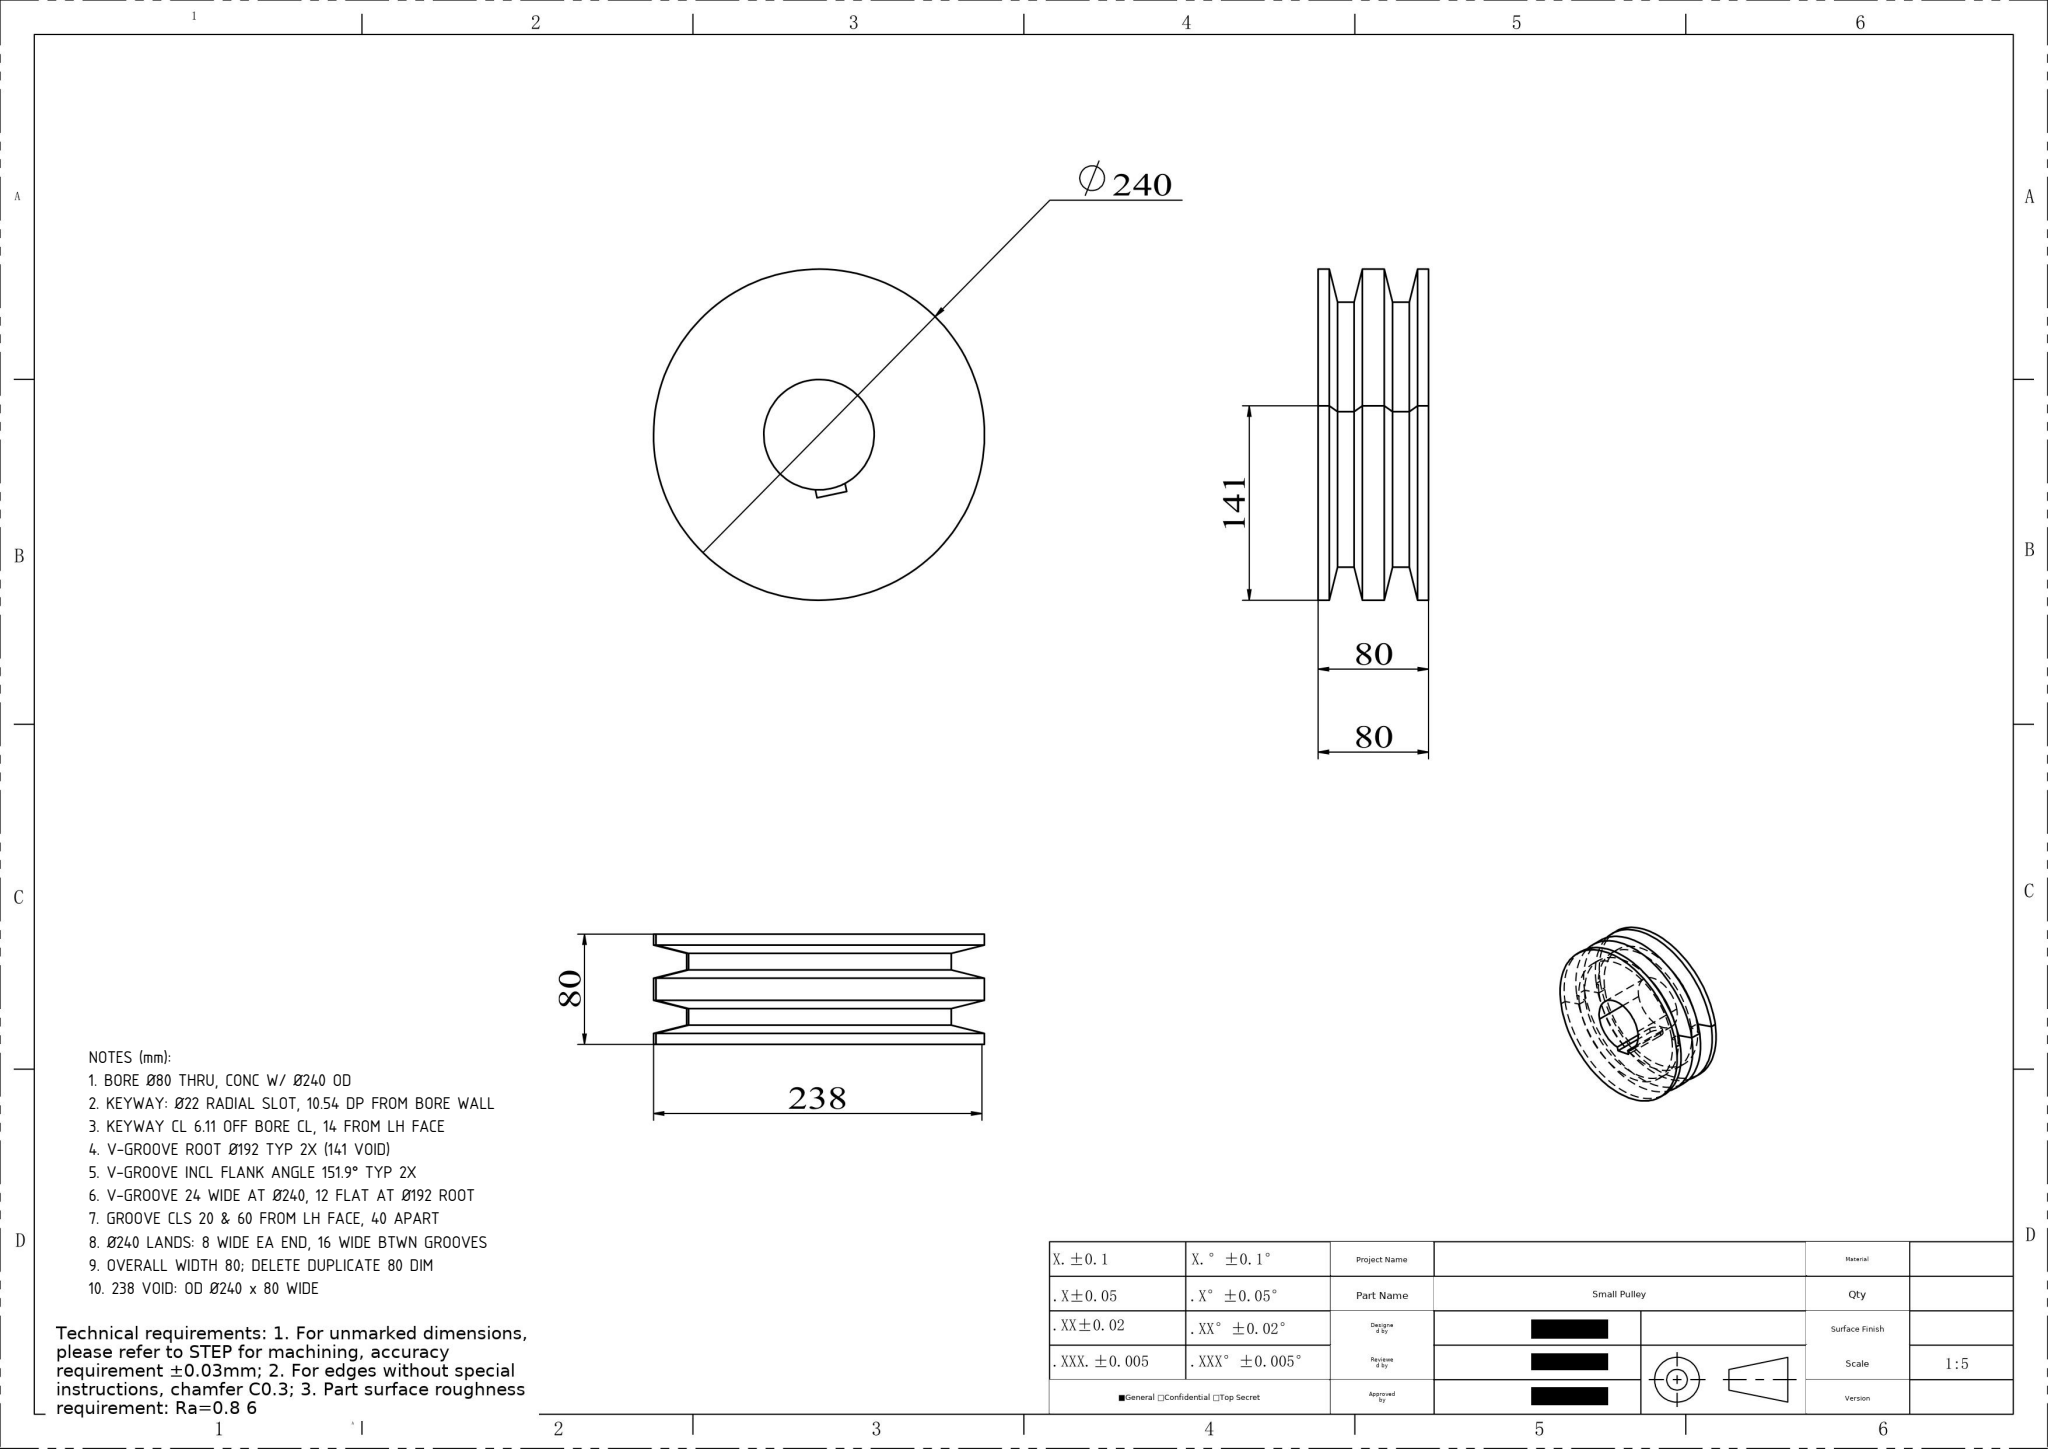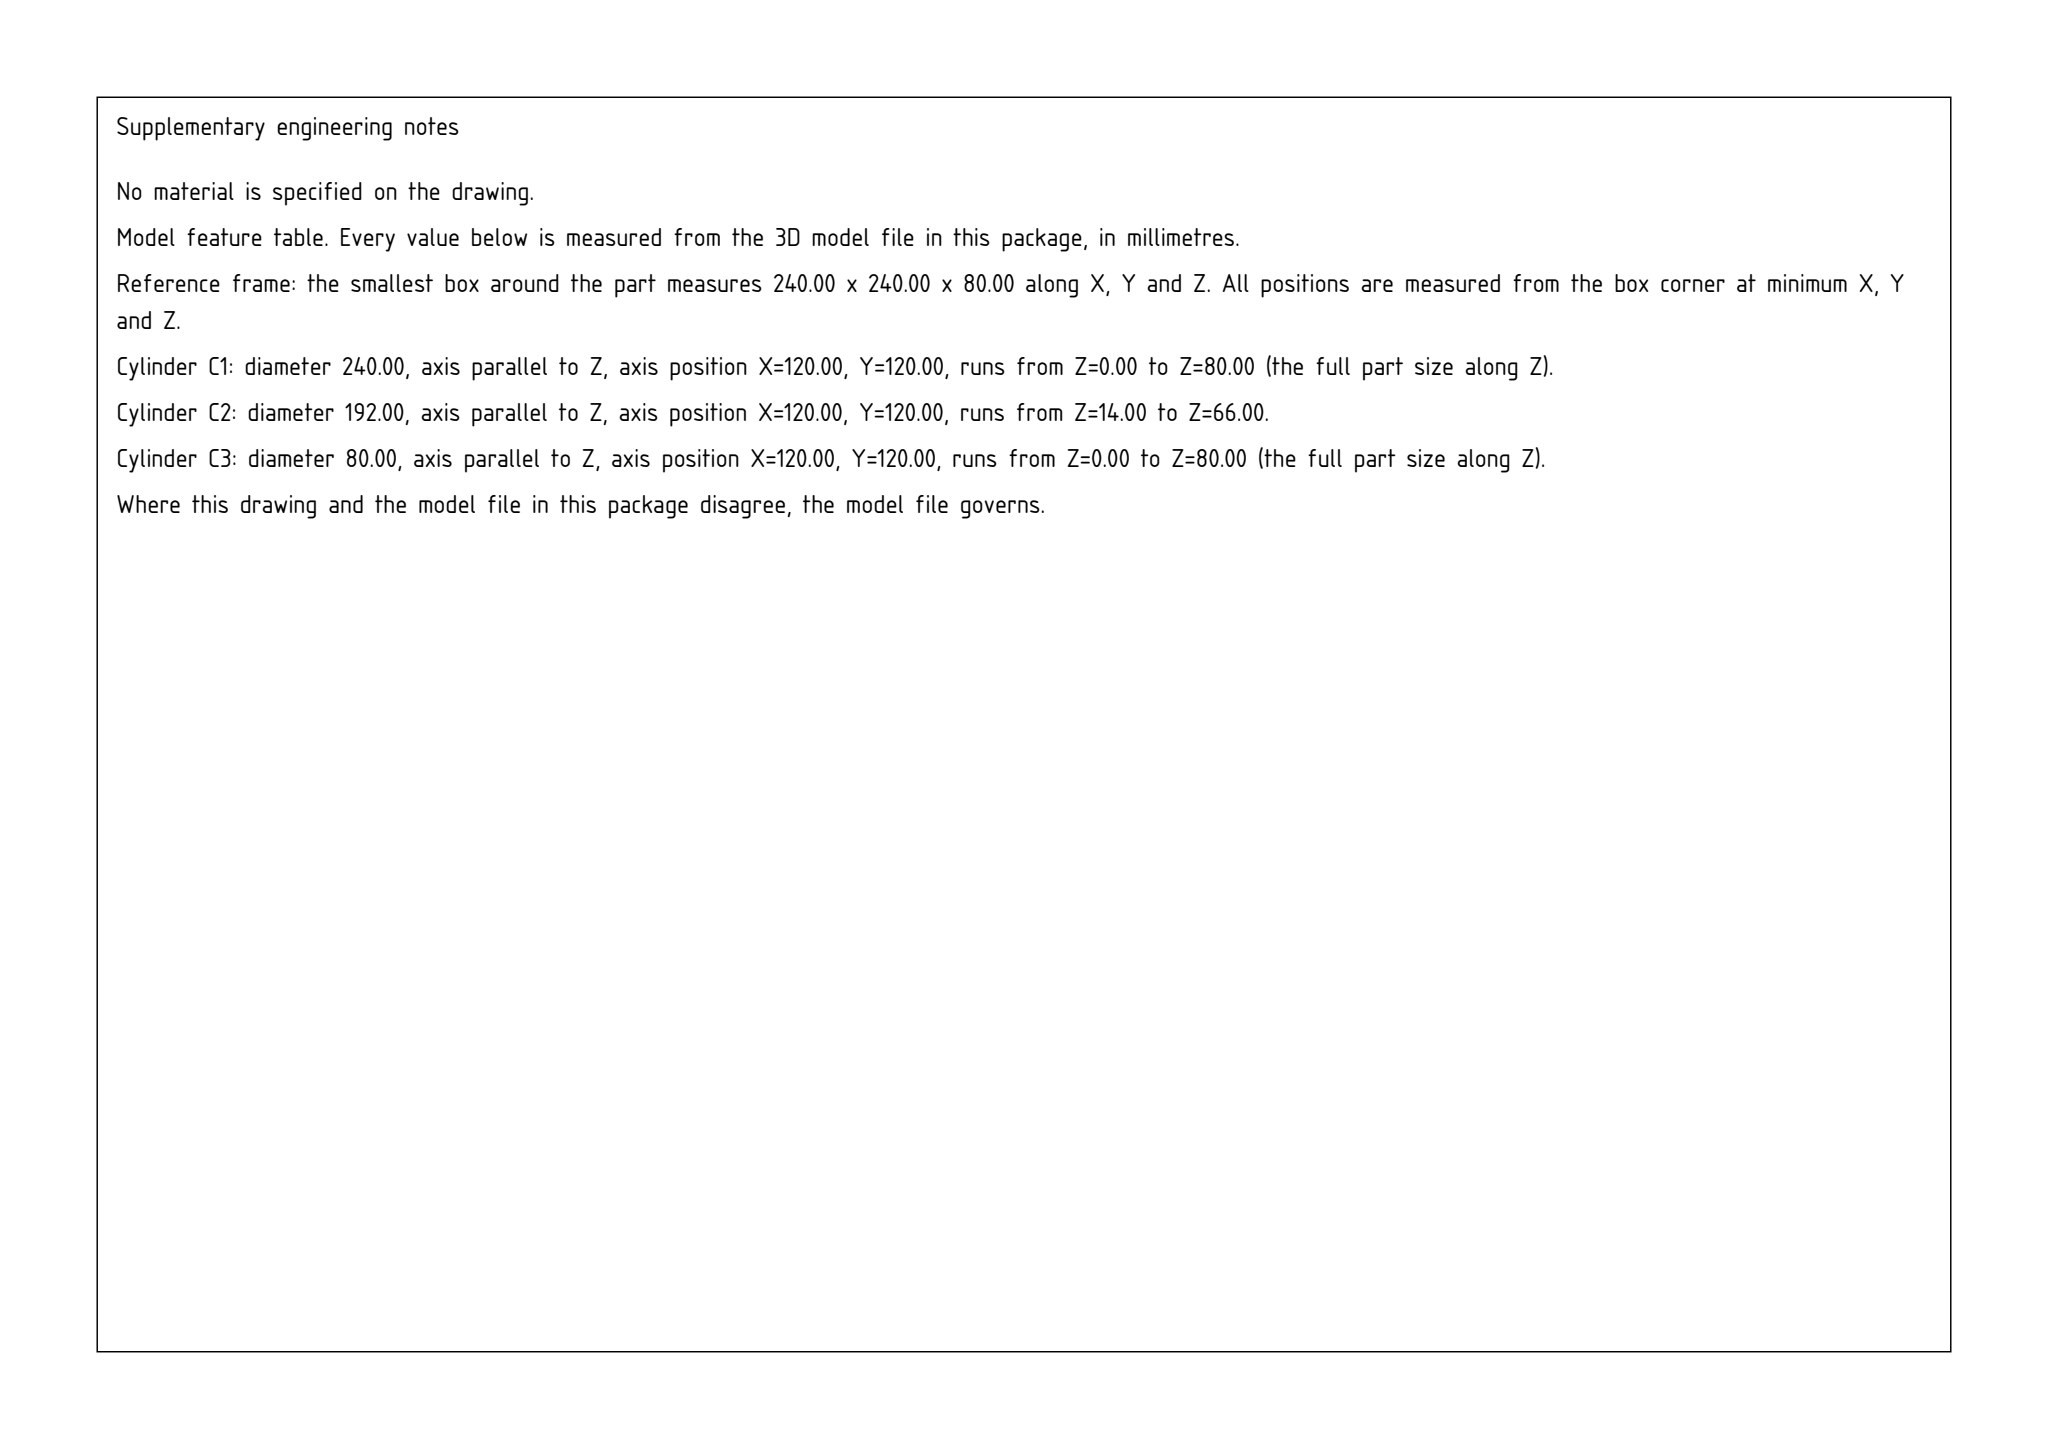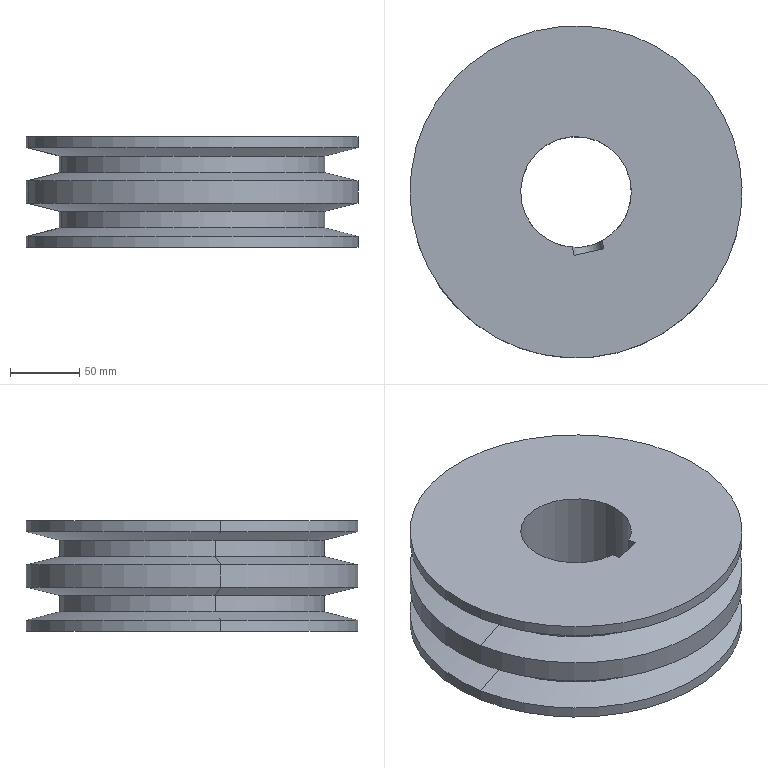Part | SolidWorks | mm | 1 solid | 26 faces | box 240 x 240 x 80 mm | volume 2615235 mm3 | cylinder 13 | cone 8 | plane 5 | commonest cylinder face diameters 240 x6 192 x4 80 x2 22 x1
Drawing notes:
BORE Ø80 THRU, CONC W/ Ø240 OD | from the solid: cyl dia 80, axis z, pos (120,120), length 80 = full width
KEYWAY: Ø22 RADIAL SLOT, 10.54 DP FROM BORE WALL | from the solid: cyl dia 22, axis y, length 10.54, breaking into Ø80 bore
KEYWAY CL 6.11 OFF BORE CL, 14 FROM LH FACE | from the solid: cyl dia22 pos x=126.11 (bore CL x=120), z=14 from z=0 face
V-GROOVE ROOT Ø192 TYP 2X (141 VOID) | from the solid: cyl dia 192, axis z, pos (120,120), length 12
V-GROOVE INCL FLANK ANGLE 151.9° TYP 2X | from the solid: cones included_angle 151.9 at ref dia 240 and 192
V-GROOVE 24 WIDE AT Ø240, 12 FLAT AT Ø192 ROOT | from the solid: Ø192 land 12 long + 2 x 6 axial flank rise (24 rad / tan75.95)
GROOVE CLS 20 & 60 FROM LH FACE, 40 APART | from the solid: grooves span z 8-32 and 48-72 within 80 wide bbox
Ø240 LANDS: 8 WIDE EA END, 16 WIDE BTWN GROOVES | from the solid: cyl dia240 lengths 8 (ends) and 16 (centre); 8+24+16+24+8=80
OVERALL WIDTH 80; DELETE DUPLICATE 80 DIM | from the solid: bbox z = 80.0, planes z=0 and z=80
238 VOID: OD Ø240 x 80 WIDE | from the solid: bbox 240 x 240 x 80; no 238 feature in model